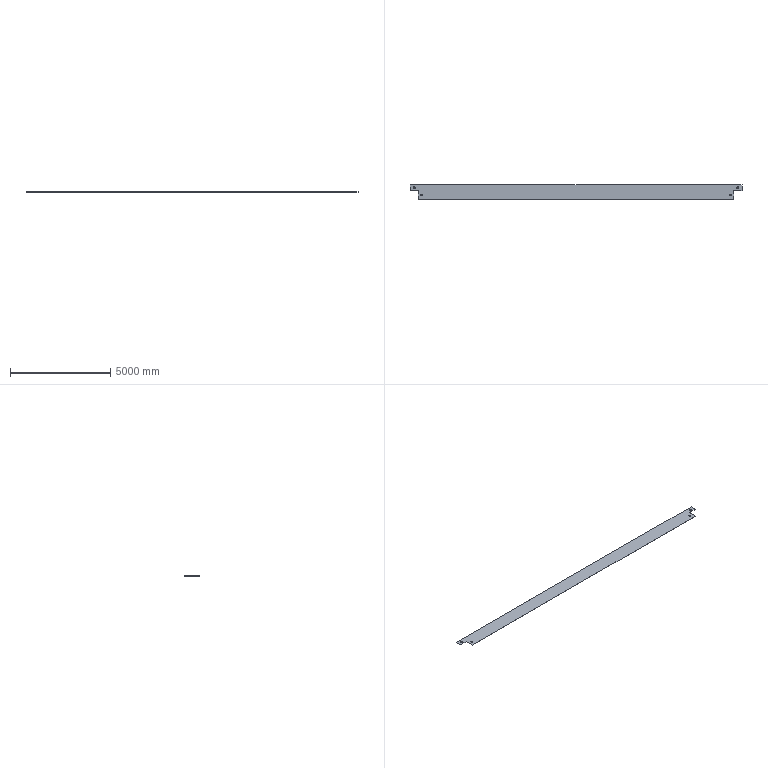Component | SolidWorks | SidePlate-1 | 1 solid | 18 faces | box 16570 x 748.03 x 6 mm | volume 70226722 mm3 | cylinder 10 | plane 8 | commonest cylinder face diameters 100 x8 3432081.25 x1 3440371.25 x1 | material Plain Carbon Steel
STEP:
#1=COLOUR_RGB('',0.7922,0.8196,0.9333);
#2=FILL_AREA_STYLE_COLOUR('',#1);
#3=FILL_AREA_STYLE('',(#2));
#4=SURFACE_STYLE_FILL_AREA(#3);
#5=SURFACE_SIDE_STYLE('',(#4));
#6=SURFACE_STYLE_USAGE(.BOTH.,#5);
#7=PRESENTATION_STYLE_ASSIGNMENT((#6));
#8=CARTESIAN_POINT('',(662.793,122.63,79.696));
#9=VERTEX_POINT('',#8);
#10=CARTESIAN_POINT('',(662.793,118.693,79.696));
#11=VERTEX_POINT('',#10);
#12=CARTESIAN_POINT('',(662.793,120.662,79.696));
#13=DIRECTION('',(0.,-0.,1.));
#14=DIRECTION('',(0.,1.,0.));
#15=AXIS2_PLACEMENT_3D('',#12,#13,#14);
#16=CIRCLE('',#15,1.969);
#17=EDGE_CURVE('',#9,#11,#16,.T.);
#18=ORIENTED_EDGE('',*,*,#17,.F.);
#19=CARTESIAN_POINT('',(662.793,122.63,79.933));
#20=VERTEX_POINT('',#19);
#21=CARTESIAN_POINT('',(662.793,122.63,79.696));
#22=DIRECTION('',(0.,-0.,1.));
#23=VECTOR('',#22,39.37);
#24=LINE('',#21,#23);
#25=EDGE_CURVE('',#9,#20,#24,.T.);
#26=ORIENTED_EDGE('',*,*,#25,.T.);
#27=CARTESIAN_POINT('',(662.793,118.693,79.933));
#28=VERTEX_POINT('',#27);
#29=CARTESIAN_POINT('',(662.793,120.662,79.933));
#30=DIRECTION('',(0.,-0.,1.));
#31=DIRECTION('',(0.,1.,0.));
#32=AXIS2_PLACEMENT_3D('',#29,#30,#31);
#33=CIRCLE('',#32,1.969);
#34=EDGE_CURVE('',#20,#28,#33,.T.);
#35=ORIENTED_EDGE('',*,*,#34,.T.);
#36=CARTESIAN_POINT('',(662.793,118.693,79.696));
#37=DIRECTION('',(0.,-0.,1.));
#38=VECTOR('',#37,39.37);
#39=LINE('',#36,#38);
#40=EDGE_CURVE('',#11,#28,#39,.T.);
#41=ORIENTED_EDGE('',*,*,#40,.F.);
#42=EDGE_LOOP('',(#18,#26,#35,#41));
#43=FACE_OUTER_BOUND('',#42,.T.);
#44=CARTESIAN_POINT('',(662.793,120.662,79.696));
#45=DIRECTION('',(0.,-0.,1.));
#46=DIRECTION('',(0.,-1.,0.));
#47=AXIS2_PLACEMENT_3D('',#44,#45,#46);
#48=CYLINDRICAL_SURFACE('',#47,1.969);
#49=ADVANCED_FACE('',(#43),#48,.F.);
#50=CARTESIAN_POINT('',(647.832,108.26,79.696));
#51=VERTEX_POINT('',#50);
#52=CARTESIAN_POINT('',(647.832,104.323,79.696));
#53=VERTEX_POINT('',#52);
#54=CARTESIAN_POINT('',(647.832,106.291,79.696));
#55=DIRECTION('',(0.,-0.,1.));
#56=DIRECTION('',(0.,1.,0.));
#57=AXIS2_PLACEMENT_3D('',#54,#55,#56);
#58=CIRCLE('',#57,1.969);
#59=EDGE_CURVE('',#51,#53,#58,.T.);
#60=ORIENTED_EDGE('',*,*,#59,.F.);
#61=CARTESIAN_POINT('',(647.832,108.26,79.933));
#62=VERTEX_POINT('',#61);
#63=CARTESIAN_POINT('',(647.832,108.26,79.696));
#64=DIRECTION('',(0.,-0.,1.));
#65=VECTOR('',#64,39.37);
#66=LINE('',#63,#65);
#67=EDGE_CURVE('',#51,#62,#66,.T.);
#68=ORIENTED_EDGE('',*,*,#67,.T.);
#69=CARTESIAN_POINT('',(647.832,104.323,79.933));
#70=VERTEX_POINT('',#69);
#71=CARTESIAN_POINT('',(647.832,106.291,79.933));
#72=DIRECTION('',(0.,-0.,1.));
#73=DIRECTION('',(0.,1.,0.));
#74=AXIS2_PLACEMENT_3D('',#71,#72,#73);
#75=CIRCLE('',#74,1.969);
#76=EDGE_CURVE('',#62,#70,#75,.T.);
#77=ORIENTED_EDGE('',*,*,#76,.T.);
#78=CARTESIAN_POINT('',(647.832,104.323,79.696));
#79=DIRECTION('',(0.,-0.,1.));
#80=VECTOR('',#79,39.37);
#81=LINE('',#78,#80);
#82=EDGE_CURVE('',#53,#70,#81,.T.);
#83=ORIENTED_EDGE('',*,*,#82,.F.);
#84=EDGE_LOOP('',(#60,#68,#77,#83));
#85=FACE_OUTER_BOUND('',#84,.T.);
#86=CARTESIAN_POINT('',(647.832,106.291,79.696));
#87=DIRECTION('',(0.,-0.,1.));
#88=DIRECTION('',(0.,-1.,0.));
#89=AXIS2_PLACEMENT_3D('',#86,#87,#88);
#90=CYLINDRICAL_SURFACE('',#89,1.969);
#91=ADVANCED_FACE('',(#85),#90,.F.);
#92=CARTESIAN_POINT('',(41.927,108.26,79.696));
#93=VERTEX_POINT('',#92);
#94=CARTESIAN_POINT('',(41.927,104.323,79.696));
#95=VERTEX_POINT('',#94);
#96=CARTESIAN_POINT('',(41.927,106.291,79.696));
#97=DIRECTION('',(0.,-0.,1.));
#98=DIRECTION('',(0.,-1.,0.));
#99=AXIS2_PLACEMENT_3D('',#96,#97,#98);
#100=CIRCLE('',#99,1.969);
#101=EDGE_CURVE('',#93,#95,#100,.T.);
#102=ORIENTED_EDGE('',*,*,#101,.F.);
#103=CARTESIAN_POINT('',(41.927,108.26,79.933));
#104=VERTEX_POINT('',#103);
#105=CARTESIAN_POINT('',(41.927,108.26,79.696));
#106=DIRECTION('',(0.,-0.,1.));
#107=VECTOR('',#106,39.37);
#108=LINE('',#105,#107);
#109=EDGE_CURVE('',#93,#104,#108,.T.);
#110=ORIENTED_EDGE('',*,*,#109,.T.);
#111=CARTESIAN_POINT('',(41.927,104.323,79.933));
#112=VERTEX_POINT('',#111);
#113=CARTESIAN_POINT('',(41.927,106.291,79.933));
#114=DIRECTION('',(0.,-0.,1.));
#115=DIRECTION('',(0.,-1.,0.));
#116=AXIS2_PLACEMENT_3D('',#113,#114,#115);
#117=CIRCLE('',#116,1.969);
#118=EDGE_CURVE('',#104,#112,#117,.T.);
#119=ORIENTED_EDGE('',*,*,#118,.T.);
#120=CARTESIAN_POINT('',(41.927,104.323,79.696));
#121=DIRECTION('',(0.,-0.,1.));
#122=VECTOR('',#121,39.37);
#123=LINE('',#120,#122);
#124=EDGE_CURVE('',#95,#112,#123,.T.);
#125=ORIENTED_EDGE('',*,*,#124,.F.);
#126=EDGE_LOOP('',(#102,#110,#119,#125));
#127=FACE_OUTER_BOUND('',#126,.T.);
#128=CARTESIAN_POINT('',(41.927,106.291,79.696));
#129=DIRECTION('',(0.,-0.,1.));
#130=DIRECTION('',(0.,-1.,0.));
#131=AXIS2_PLACEMENT_3D('',#128,#129,#130);
#132=CYLINDRICAL_SURFACE('',#131,1.969);
#133=ADVANCED_FACE('',(#127),#132,.F.);
#134=CARTESIAN_POINT('',(26.966,122.63,79.696));
#135=VERTEX_POINT('',#134);
#136=CARTESIAN_POINT('',(26.966,118.693,79.696));
#137=VERTEX_POINT('',#136);
#138=CARTESIAN_POINT('',(26.966,120.662,79.696));
#139=DIRECTION('',(0.,-0.,1.));
#140=DIRECTION('',(0.,-1.,0.));
#141=AXIS2_PLACEMENT_3D('',#138,#139,#140);
#142=CIRCLE('',#141,1.969);
#143=EDGE_CURVE('',#135,#137,#142,.T.);
#144=ORIENTED_EDGE('',*,*,#143,.F.);
#145=CARTESIAN_POINT('',(26.966,122.63,79.933));
#146=VERTEX_POINT('',#145);
#147=CARTESIAN_POINT('',(26.966,122.63,79.696));
#148=DIRECTION('',(0.,-0.,1.));
#149=VECTOR('',#148,39.37);
#150=LINE('',#147,#149);
#151=EDGE_CURVE('',#135,#146,#150,.T.);
#152=ORIENTED_EDGE('',*,*,#151,.T.);
#153=CARTESIAN_POINT('',(26.966,118.693,79.933));
#154=VERTEX_POINT('',#153);
#155=CARTESIAN_POINT('',(26.966,120.662,79.933));
#156=DIRECTION('',(0.,-0.,1.));
#157=DIRECTION('',(0.,-1.,0.));
#158=AXIS2_PLACEMENT_3D('',#155,#156,#157);
#159=CIRCLE('',#158,1.969);
#160=EDGE_CURVE('',#146,#154,#159,.T.);
#161=ORIENTED_EDGE('',*,*,#160,.T.);
#162=CARTESIAN_POINT('',(26.966,118.693,79.696));
#163=DIRECTION('',(0.,-0.,1.));
#164=VECTOR('',#163,39.37);
#165=LINE('',#162,#164);
#166=EDGE_CURVE('',#137,#154,#165,.T.);
#167=ORIENTED_EDGE('',*,*,#166,.F.);
#168=EDGE_LOOP('',(#144,#152,#161,#167));
#169=FACE_OUTER_BOUND('',#168,.T.);
#170=CARTESIAN_POINT('',(26.966,120.662,79.696));
#171=DIRECTION('',(0.,-0.,1.));
#172=DIRECTION('',(0.,-1.,0.));
#173=AXIS2_PLACEMENT_3D('',#170,#171,#172);
#174=CYLINDRICAL_SURFACE('',#173,1.969);
#175=ADVANCED_FACE('',(#169),#174,.F.);
#176=CARTESIAN_POINT('',(671.061,126.37,79.933));
#177=VERTEX_POINT('',#176);
#178=CARTESIAN_POINT('',(18.698,126.37,79.933));
#179=VERTEX_POINT('',#178);
#180=CARTESIAN_POINT('',(344.879,-67433.497,79.933));
#181=DIRECTION('',(0.,-0.,1.));
#182=DIRECTION('',(0.,1.,0.));
#183=AXIS2_PLACEMENT_3D('',#180,#181,#182);
#184=CIRCLE('',#183,67560.655);
#185=EDGE_CURVE('',#177,#179,#184,.T.);
#186=ORIENTED_EDGE('',*,*,#185,.F.);
#187=CARTESIAN_POINT('',(671.061,126.37,79.696));
#188=VERTEX_POINT('',#187);
#189=CARTESIAN_POINT('',(671.061,126.37,79.696));
#190=DIRECTION('',(0.,-0.,1.));
#191=VECTOR('',#190,39.37);
#192=LINE('',#189,#191);
#193=EDGE_CURVE('',#188,#177,#192,.T.);
#194=ORIENTED_EDGE('',*,*,#193,.F.);
#195=CARTESIAN_POINT('',(18.698,126.37,79.696));
#196=VERTEX_POINT('',#195);
#197=CARTESIAN_POINT('',(344.879,-67433.497,79.696));
#198=DIRECTION('',(0.,-0.,1.));
#199=DIRECTION('',(0.,1.,0.));
#200=AXIS2_PLACEMENT_3D('',#197,#198,#199);
#201=CIRCLE('',#200,67560.655);
#202=EDGE_CURVE('',#188,#196,#201,.T.);
#203=ORIENTED_EDGE('',*,*,#202,.T.);
#204=CARTESIAN_POINT('',(18.698,126.37,79.696));
#205=DIRECTION('',(0.,-0.,1.));
#206=VECTOR('',#205,39.37);
#207=LINE('',#204,#206);
#208=EDGE_CURVE('',#196,#179,#207,.T.);
#209=ORIENTED_EDGE('',*,*,#208,.T.);
#210=EDGE_LOOP('',(#186,#194,#203,#209));
#211=FACE_OUTER_BOUND('',#210,.T.);
#212=CARTESIAN_POINT('',(344.879,-67433.497,79.696));
#213=DIRECTION('',(0.,-0.,1.));
#214=DIRECTION('',(0.,-1.,-0.));
#215=AXIS2_PLACEMENT_3D('',#212,#213,#214);
#216=CYLINDRICAL_SURFACE('',#215,67560.655);
#217=ADVANCED_FACE('',(#211),#216,.T.);
#218=CARTESIAN_POINT('',(671.061,114.953,79.933));
#219=VERTEX_POINT('',#218);
#220=CARTESIAN_POINT('',(671.061,114.953,79.933));
#221=DIRECTION('',(0.,1.,0.));
#222=VECTOR('',#221,39.37);
#223=LINE('',#220,#222);
#224=EDGE_CURVE('',#219,#177,#223,.T.);
#225=ORIENTED_EDGE('',*,*,#224,.F.);
#226=CARTESIAN_POINT('',(671.061,114.953,79.696));
#227=VERTEX_POINT('',#226);
#228=CARTESIAN_POINT('',(671.061,114.953,79.696));
#229=DIRECTION('',(0.,-0.,1.));
#230=VECTOR('',#229,39.37);
#231=LINE('',#228,#230);
#232=EDGE_CURVE('',#227,#219,#231,.T.);
#233=ORIENTED_EDGE('',*,*,#232,.F.);
#234=CARTESIAN_POINT('',(671.061,114.953,79.696));
#235=DIRECTION('',(0.,1.,0.));
#236=VECTOR('',#235,39.37);
#237=LINE('',#234,#236);
#238=EDGE_CURVE('',#227,#188,#237,.T.);
#239=ORIENTED_EDGE('',*,*,#238,.T.);
#240=ORIENTED_EDGE('',*,*,#193,.T.);
#241=EDGE_LOOP('',(#225,#233,#239,#240));
#242=FACE_OUTER_BOUND('',#241,.T.);
#243=CARTESIAN_POINT('',(671.061,114.953,79.696));
#244=DIRECTION('',(1.,0.,0.));
#245=DIRECTION('',(0.,1.,0.));
#246=AXIS2_PLACEMENT_3D('',#243,#244,#245);
#247=PLANE('',#246);
#248=ADVANCED_FACE('',(#242),#247,.T.);
#249=CARTESIAN_POINT('',(654.919,114.953,79.933));
#250=VERTEX_POINT('',#249);
#251=CARTESIAN_POINT('',(671.061,114.953,79.933));
#252=DIRECTION('',(1.,0.,0.));
#253=VECTOR('',#252,39.37);
#254=LINE('',#251,#253);
#255=EDGE_CURVE('',#250,#219,#254,.T.);
#256=ORIENTED_EDGE('',*,*,#255,.F.);
#257=CARTESIAN_POINT('',(654.919,114.953,79.696));
#258=VERTEX_POINT('',#257);
#259=CARTESIAN_POINT('',(654.919,114.953,79.696));
#260=DIRECTION('',(0.,-0.,1.));
#261=VECTOR('',#260,39.37);
#262=LINE('',#259,#261);
#263=EDGE_CURVE('',#258,#250,#262,.T.);
#264=ORIENTED_EDGE('',*,*,#263,.F.);
#265=CARTESIAN_POINT('',(671.061,114.953,79.696));
#266=DIRECTION('',(1.,0.,0.));
#267=VECTOR('',#266,39.37);
#268=LINE('',#265,#267);
#269=EDGE_CURVE('',#258,#227,#268,.T.);
#270=ORIENTED_EDGE('',*,*,#269,.T.);
#271=ORIENTED_EDGE('',*,*,#232,.T.);
#272=EDGE_LOOP('',(#256,#264,#270,#271));
#273=FACE_OUTER_BOUND('',#272,.T.);
#274=CARTESIAN_POINT('',(671.061,114.953,79.696));
#275=DIRECTION('',(0.,-1.,-0.));
#276=DIRECTION('',(1.,0.,0.));
#277=AXIS2_PLACEMENT_3D('',#274,#275,#276);
#278=PLANE('',#277);
#279=ADVANCED_FACE('',(#273),#278,.T.);
#280=CARTESIAN_POINT('',(654.919,97.708,79.933));
#281=VERTEX_POINT('',#280);
#282=CARTESIAN_POINT('',(654.919,114.953,79.933));
#283=DIRECTION('',(0.,1.,0.));
#284=VECTOR('',#283,39.37);
#285=LINE('',#282,#284);
#286=EDGE_CURVE('',#281,#250,#285,.T.);
#287=ORIENTED_EDGE('',*,*,#286,.F.);
#288=CARTESIAN_POINT('',(654.919,97.708,79.696));
#289=VERTEX_POINT('',#288);
#290=CARTESIAN_POINT('',(654.919,97.708,79.696));
#291=DIRECTION('',(0.,-0.,1.));
#292=VECTOR('',#291,39.37);
#293=LINE('',#290,#292);
#294=EDGE_CURVE('',#289,#281,#293,.T.);
#295=ORIENTED_EDGE('',*,*,#294,.F.);
#296=CARTESIAN_POINT('',(654.919,114.953,79.696));
#297=DIRECTION('',(0.,1.,0.));
#298=VECTOR('',#297,39.37);
#299=LINE('',#296,#298);
#300=EDGE_CURVE('',#289,#258,#299,.T.);
#301=ORIENTED_EDGE('',*,*,#300,.T.);
#302=ORIENTED_EDGE('',*,*,#263,.T.);
#303=EDGE_LOOP('',(#287,#295,#301,#302));
#304=FACE_OUTER_BOUND('',#303,.T.);
#305=CARTESIAN_POINT('',(654.919,114.953,79.696));
#306=DIRECTION('',(1.,0.,0.));
#307=DIRECTION('',(0.,1.,0.));
#308=AXIS2_PLACEMENT_3D('',#305,#306,#307);
#309=PLANE('',#308);
#310=ADVANCED_FACE('',(#304),#309,.T.);
#311=CARTESIAN_POINT('',(34.84,97.708,79.933));
#312=VERTEX_POINT('',#311);
#313=CARTESIAN_POINT('',(344.879,-67625.426,79.933));
#314=DIRECTION('',(0.,0.,-1.));
#315=DIRECTION('',(0.,1.,0.));
#316=AXIS2_PLACEMENT_3D('',#313,#314,#315);
#317=CIRCLE('',#316,67723.844);
#318=EDGE_CURVE('',#312,#281,#317,.T.);
#319=ORIENTED_EDGE('',*,*,#318,.F.);
#320=CARTESIAN_POINT('',(34.84,97.708,79.696));
#321=VERTEX_POINT('',#320);
#322=CARTESIAN_POINT('',(34.84,97.708,79.696));
#323=DIRECTION('',(0.,-0.,1.));
#324=VECTOR('',#323,39.37);
#325=LINE('',#322,#324);
#326=EDGE_CURVE('',#321,#312,#325,.T.);
#327=ORIENTED_EDGE('',*,*,#326,.F.);
#328=CARTESIAN_POINT('',(344.879,-67625.426,79.696));
#329=DIRECTION('',(0.,0.,-1.));
#330=DIRECTION('',(0.,1.,0.));
#331=AXIS2_PLACEMENT_3D('',#328,#329,#330);
#332=CIRCLE('',#331,67723.844);
#333=EDGE_CURVE('',#321,#289,#332,.T.);
#334=ORIENTED_EDGE('',*,*,#333,.T.);
#335=ORIENTED_EDGE('',*,*,#294,.T.);
#336=EDGE_LOOP('',(#319,#327,#334,#335));
#337=FACE_OUTER_BOUND('',#336,.T.);
#338=CARTESIAN_POINT('',(344.879,-67625.426,79.696));
#339=DIRECTION('',(0.,-0.,1.));
#340=DIRECTION('',(0.,-1.,-0.));
#341=AXIS2_PLACEMENT_3D('',#338,#339,#340);
#342=CYLINDRICAL_SURFACE('',#341,67723.844);
#343=ADVANCED_FACE('',(#337),#342,.F.);
#344=CARTESIAN_POINT('',(34.84,114.953,79.933));
#345=VERTEX_POINT('',#344);
#346=CARTESIAN_POINT('',(34.84,114.953,79.933));
#347=DIRECTION('',(0.,-1.,-0.));
#348=VECTOR('',#347,39.37);
#349=LINE('',#346,#348);
#350=EDGE_CURVE('',#345,#312,#349,.T.);
#351=ORIENTED_EDGE('',*,*,#350,.F.);
#352=CARTESIAN_POINT('',(34.84,114.953,79.696));
#353=VERTEX_POINT('',#352);
#354=CARTESIAN_POINT('',(34.84,114.953,79.696));
#355=DIRECTION('',(0.,-0.,1.));
#356=VECTOR('',#355,39.37);
#357=LINE('',#354,#356);
#358=EDGE_CURVE('',#353,#345,#357,.T.);
#359=ORIENTED_EDGE('',*,*,#358,.F.);
#360=CARTESIAN_POINT('',(34.84,114.953,79.696));
#361=DIRECTION('',(0.,-1.,-0.));
#362=VECTOR('',#361,39.37);
#363=LINE('',#360,#362);
#364=EDGE_CURVE('',#353,#321,#363,.T.);
#365=ORIENTED_EDGE('',*,*,#364,.T.);
#366=ORIENTED_EDGE('',*,*,#326,.T.);
#367=EDGE_LOOP('',(#351,#359,#365,#366));
#368=FACE_OUTER_BOUND('',#367,.T.);
#369=CARTESIAN_POINT('',(34.84,114.953,79.696));
#370=DIRECTION('',(-1.,-0.,-0.));
#371=DIRECTION('',(0.,-1.,-0.));
#372=AXIS2_PLACEMENT_3D('',#369,#370,#371);
#373=PLANE('',#372);
#374=ADVANCED_FACE('',(#368),#373,.T.);
#375=CARTESIAN_POINT('',(18.698,114.953,79.933));
#376=VERTEX_POINT('',#375);
#377=CARTESIAN_POINT('',(18.698,114.953,79.933));
#378=DIRECTION('',(1.,0.,0.));
#379=VECTOR('',#378,39.37);
#380=LINE('',#377,#379);
#381=EDGE_CURVE('',#376,#345,#380,.T.);
#382=ORIENTED_EDGE('',*,*,#381,.F.);
#383=CARTESIAN_POINT('',(18.698,114.953,79.696));
#384=VERTEX_POINT('',#383);
#385=CARTESIAN_POINT('',(18.698,114.953,79.696));
#386=DIRECTION('',(0.,-0.,1.));
#387=VECTOR('',#386,39.37);
#388=LINE('',#385,#387);
#389=EDGE_CURVE('',#384,#376,#388,.T.);
#390=ORIENTED_EDGE('',*,*,#389,.F.);
#391=CARTESIAN_POINT('',(18.698,114.953,79.696));
#392=DIRECTION('',(1.,0.,0.));
#393=VECTOR('',#392,39.37);
#394=LINE('',#391,#393);
#395=EDGE_CURVE('',#384,#353,#394,.T.);
#396=ORIENTED_EDGE('',*,*,#395,.T.);
#397=ORIENTED_EDGE('',*,*,#358,.T.);
#398=EDGE_LOOP('',(#382,#390,#396,#397));
#399=FACE_OUTER_BOUND('',#398,.T.);
#400=CARTESIAN_POINT('',(18.698,114.953,79.696));
#401=DIRECTION('',(0.,-1.,-0.));
#402=DIRECTION('',(1.,0.,0.));
#403=AXIS2_PLACEMENT_3D('',#400,#401,#402);
#404=PLANE('',#403);
#405=ADVANCED_FACE('',(#399),#404,.T.);
#406=CARTESIAN_POINT('',(18.698,126.37,79.933));
#407=DIRECTION('',(0.,-1.,-0.));
#408=VECTOR('',#407,39.37);
#409=LINE('',#406,#408);
#410=EDGE_CURVE('',#179,#376,#409,.T.);
#411=ORIENTED_EDGE('',*,*,#410,.F.);
#412=ORIENTED_EDGE('',*,*,#208,.F.);
#413=CARTESIAN_POINT('',(18.698,126.37,79.696));
#414=DIRECTION('',(0.,-1.,-0.));
#415=VECTOR('',#414,39.37);
#416=LINE('',#413,#415);
#417=EDGE_CURVE('',#196,#384,#416,.T.);
#418=ORIENTED_EDGE('',*,*,#417,.T.);
#419=ORIENTED_EDGE('',*,*,#389,.T.);
#420=EDGE_LOOP('',(#411,#412,#418,#419));
#421=FACE_OUTER_BOUND('',#420,.T.);
#422=CARTESIAN_POINT('',(18.698,126.37,79.696));
#423=DIRECTION('',(-1.,-0.,-0.));
#424=DIRECTION('',(0.,-1.,-0.));
#425=AXIS2_PLACEMENT_3D('',#422,#423,#424);
#426=PLANE('',#425);
#427=ADVANCED_FACE('',(#421),#426,.T.);
#428=CARTESIAN_POINT('',(662.793,120.662,79.696));
#429=DIRECTION('',(0.,-0.,1.));
#430=DIRECTION('',(0.,1.,0.));
#431=AXIS2_PLACEMENT_3D('',#428,#429,#430);
#432=CIRCLE('',#431,1.969);
#433=EDGE_CURVE('',#11,#9,#432,.T.);
#434=ORIENTED_EDGE('',*,*,#433,.T.);
#435=ORIENTED_EDGE('',*,*,#17,.T.);
#436=EDGE_LOOP('',(#434,#435));
#437=FACE_BOUND('',#436,.T.);
#438=CARTESIAN_POINT('',(647.832,106.291,79.696));
#439=DIRECTION('',(0.,-0.,1.));
#440=DIRECTION('',(0.,1.,0.));
#441=AXIS2_PLACEMENT_3D('',#438,#439,#440);
#442=CIRCLE('',#441,1.969);
#443=EDGE_CURVE('',#53,#51,#442,.T.);
#444=ORIENTED_EDGE('',*,*,#443,.T.);
#445=ORIENTED_EDGE('',*,*,#59,.T.);
#446=EDGE_LOOP('',(#444,#445));
#447=FACE_BOUND('',#446,.T.);
#448=CARTESIAN_POINT('',(41.927,106.291,79.696));
#449=DIRECTION('',(0.,-0.,1.));
#450=DIRECTION('',(0.,-1.,0.));
#451=AXIS2_PLACEMENT_3D('',#448,#449,#450);
#452=CIRCLE('',#451,1.969);
#453=EDGE_CURVE('',#95,#93,#452,.T.);
#454=ORIENTED_EDGE('',*,*,#453,.T.);
#455=ORIENTED_EDGE('',*,*,#101,.T.);
#456=EDGE_LOOP('',(#454,#455));
#457=FACE_BOUND('',#456,.T.);
#458=CARTESIAN_POINT('',(26.966,120.662,79.696));
#459=DIRECTION('',(0.,-0.,1.));
#460=DIRECTION('',(0.,-1.,0.));
#461=AXIS2_PLACEMENT_3D('',#458,#459,#460);
#462=CIRCLE('',#461,1.969);
#463=EDGE_CURVE('',#137,#135,#462,.T.);
#464=ORIENTED_EDGE('',*,*,#463,.T.);
#465=ORIENTED_EDGE('',*,*,#143,.T.);
#466=EDGE_LOOP('',(#464,#465));
#467=FACE_BOUND('',#466,.T.);
#468=ORIENTED_EDGE('',*,*,#202,.F.);
#469=ORIENTED_EDGE('',*,*,#238,.F.);
#470=ORIENTED_EDGE('',*,*,#269,.F.);
#471=ORIENTED_EDGE('',*,*,#300,.F.);
#472=ORIENTED_EDGE('',*,*,#333,.F.);
#473=ORIENTED_EDGE('',*,*,#364,.F.);
#474=ORIENTED_EDGE('',*,*,#395,.F.);
#475=ORIENTED_EDGE('',*,*,#417,.F.);
#476=EDGE_LOOP('',(#468,#469,#470,#471,#472,#473,#474,#475));
#477=FACE_OUTER_BOUND('',#476,.T.);
#478=CARTESIAN_POINT('',(344.879,-67433.497,79.696));
#479=DIRECTION('',(0.,0.,-1.));
#480=DIRECTION('',(0.,1.,0.));
#481=AXIS2_PLACEMENT_3D('',#478,#479,#480);
#482=PLANE('',#481);
#483=ADVANCED_FACE('',(#437,#447,#457,#467,#477),#482,.T.);
#484=CARTESIAN_POINT('',(662.793,120.662,79.933));
#485=DIRECTION('',(0.,-0.,1.));
#486=DIRECTION('',(0.,1.,0.));
#487=AXIS2_PLACEMENT_3D('',#484,#485,#486);
#488=CIRCLE('',#487,1.969);
#489=EDGE_CURVE('',#28,#20,#488,.T.);
#490=ORIENTED_EDGE('',*,*,#489,.F.);
#491=ORIENTED_EDGE('',*,*,#34,.F.);
#492=EDGE_LOOP('',(#490,#491));
#493=FACE_BOUND('',#492,.T.);
#494=CARTESIAN_POINT('',(647.832,106.291,79.933));
#495=DIRECTION('',(0.,-0.,1.));
#496=DIRECTION('',(0.,1.,0.));
#497=AXIS2_PLACEMENT_3D('',#494,#495,#496);
#498=CIRCLE('',#497,1.969);
#499=EDGE_CURVE('',#70,#62,#498,.T.);
#500=ORIENTED_EDGE('',*,*,#499,.F.);
#501=ORIENTED_EDGE('',*,*,#76,.F.);
#502=EDGE_LOOP('',(#500,#501));
#503=FACE_BOUND('',#502,.T.);
#504=CARTESIAN_POINT('',(41.927,106.291,79.933));
#505=DIRECTION('',(0.,-0.,1.));
#506=DIRECTION('',(0.,-1.,0.));
#507=AXIS2_PLACEMENT_3D('',#504,#505,#506);
#508=CIRCLE('',#507,1.969);
#509=EDGE_CURVE('',#112,#104,#508,.T.);
#510=ORIENTED_EDGE('',*,*,#509,.F.);
#511=ORIENTED_EDGE('',*,*,#118,.F.);
#512=EDGE_LOOP('',(#510,#511));
#513=FACE_BOUND('',#512,.T.);
#514=CARTESIAN_POINT('',(26.966,120.662,79.933));
#515=DIRECTION('',(0.,-0.,1.));
#516=DIRECTION('',(0.,-1.,0.));
#517=AXIS2_PLACEMENT_3D('',#514,#515,#516);
#518=CIRCLE('',#517,1.969);
#519=EDGE_CURVE('',#154,#146,#518,.T.);
#520=ORIENTED_EDGE('',*,*,#519,.F.);
#521=ORIENTED_EDGE('',*,*,#160,.F.);
#522=EDGE_LOOP('',(#520,#521));
#523=FACE_BOUND('',#522,.T.);
#524=ORIENTED_EDGE('',*,*,#185,.T.);
#525=ORIENTED_EDGE('',*,*,#410,.T.);
#526=ORIENTED_EDGE('',*,*,#381,.T.);
#527=ORIENTED_EDGE('',*,*,#350,.T.);
#528=ORIENTED_EDGE('',*,*,#318,.T.);
#529=ORIENTED_EDGE('',*,*,#286,.T.);
#530=ORIENTED_EDGE('',*,*,#255,.T.);
#531=ORIENTED_EDGE('',*,*,#224,.T.);
#532=EDGE_LOOP('',(#524,#525,#526,#527,#528,#529,#530,#531));
#533=FACE_OUTER_BOUND('',#532,.T.);
#534=CARTESIAN_POINT('',(344.879,-67433.497,79.933));
#535=DIRECTION('',(0.,0.,-1.));
#536=DIRECTION('',(0.,1.,0.));
#537=AXIS2_PLACEMENT_3D('',#534,#535,#536);
#538=PLANE('',#537);
#539=ADVANCED_FACE('',(#493,#503,#513,#523,#533),#538,.F.);
#540=ORIENTED_EDGE('',*,*,#151,.F.);
#541=ORIENTED_EDGE('',*,*,#463,.F.);
#542=ORIENTED_EDGE('',*,*,#166,.T.);
#543=ORIENTED_EDGE('',*,*,#519,.T.);
#544=EDGE_LOOP('',(#540,#541,#542,#543));
#545=FACE_OUTER_BOUND('',#544,.T.);
#546=CARTESIAN_POINT('',(26.966,120.662,79.696));
#547=DIRECTION('',(0.,-0.,1.));
#548=DIRECTION('',(0.,-1.,0.));
#549=AXIS2_PLACEMENT_3D('',#546,#547,#548);
#550=CYLINDRICAL_SURFACE('',#549,1.969);
#551=ADVANCED_FACE('',(#545),#550,.F.);
#552=ORIENTED_EDGE('',*,*,#109,.F.);
#553=ORIENTED_EDGE('',*,*,#453,.F.);
#554=ORIENTED_EDGE('',*,*,#124,.T.);
#555=ORIENTED_EDGE('',*,*,#509,.T.);
#556=EDGE_LOOP('',(#552,#553,#554,#555));
#557=FACE_OUTER_BOUND('',#556,.T.);
#558=CARTESIAN_POINT('',(41.927,106.291,79.696));
#559=DIRECTION('',(0.,-0.,1.));
#560=DIRECTION('',(0.,-1.,0.));
#561=AXIS2_PLACEMENT_3D('',#558,#559,#560);
#562=CYLINDRICAL_SURFACE('',#561,1.969);
#563=ADVANCED_FACE('',(#557),#562,.F.);
#564=ORIENTED_EDGE('',*,*,#67,.F.);
#565=ORIENTED_EDGE('',*,*,#443,.F.);
#566=ORIENTED_EDGE('',*,*,#82,.T.);
#567=ORIENTED_EDGE('',*,*,#499,.T.);
#568=EDGE_LOOP('',(#564,#565,#566,#567));
#569=FACE_OUTER_BOUND('',#568,.T.);
#570=CARTESIAN_POINT('',(647.832,106.291,79.696));
#571=DIRECTION('',(0.,-0.,1.));
#572=DIRECTION('',(0.,-1.,0.));
#573=AXIS2_PLACEMENT_3D('',#570,#571,#572);
#574=CYLINDRICAL_SURFACE('',#573,1.969);
#575=ADVANCED_FACE('',(#569),#574,.F.);
#576=ORIENTED_EDGE('',*,*,#25,.F.);
#577=ORIENTED_EDGE('',*,*,#433,.F.);
#578=ORIENTED_EDGE('',*,*,#40,.T.);
#579=ORIENTED_EDGE('',*,*,#489,.T.);
#580=EDGE_LOOP('',(#576,#577,#578,#579));
#581=FACE_OUTER_BOUND('',#580,.T.);
#582=CARTESIAN_POINT('',(662.793,120.662,79.696));
#583=DIRECTION('',(0.,-0.,1.));
#584=DIRECTION('',(0.,-1.,0.));
#585=AXIS2_PLACEMENT_3D('',#582,#583,#584);
#586=CYLINDRICAL_SURFACE('',#585,1.969);
#587=ADVANCED_FACE('',(#581),#586,.F.);
#588=CLOSED_SHELL('',(#49,#91,#133,#175,#217,#248,#279,#310,#343,#374,#405,#427,#483,#539,#551,#563,#575,#587));
#589=MANIFOLD_SOLID_BREP('',#588);
#590=STYLED_ITEM('',(#7),#589);
#591=PRESENTATION_LAYER_ASSIGNMENT('','',(#590));
#592=CARTESIAN_POINT('',(0.,0.,0.));
#593=DIRECTION('',(0.,0.,1.));
#594=DIRECTION('',(1.,0.,0.));
#595=AXIS2_PLACEMENT_3D('',#592,#593,#594);
#596=(LENGTH_UNIT()NAMED_UNIT(*)SI_UNIT($,.METRE.));
#597=LENGTH_MEASURE_WITH_UNIT(LENGTH_MEASURE(0.0254),#596);
#598=DIMENSIONAL_EXPONENTS(1.,0.,0.,0.,0.,0.,0.);
#599=(CONVERSION_BASED_UNIT('',#597)LENGTH_UNIT()NAMED_UNIT(#598));
#600=UNCERTAINTY_MEASURE_WITH_UNIT(LENGTH_MEASURE(0.00001),#599,'','');
#601=(NAMED_UNIT(*)PLANE_ANGLE_UNIT()SI_UNIT($,.RADIAN.));
#602=(NAMED_UNIT(*)SI_UNIT($,.STERADIAN.)SOLID_ANGLE_UNIT());
#603=(GEOMETRIC_REPRESENTATION_CONTEXT(3)GLOBAL_UNCERTAINTY_ASSIGNED_CONTEXT((#600))GLOBAL_UNIT_ASSIGNED_CONTEXT((#599,#601,#602))REPRESENTATION_CONTEXT('',''));
#604=ADVANCED_BREP_SHAPE_REPRESENTATION('',(#589,#595),#603);
#605=(LENGTH_UNIT()NAMED_UNIT(*)SI_UNIT($,.METRE.));
#606=LENGTH_MEASURE_WITH_UNIT(LENGTH_MEASURE(0.0254),#605);
#607=DIMENSIONAL_EXPONENTS(1.,0.,0.,0.,0.,0.,0.);
#608=(CONVERSION_BASED_UNIT('',#606)LENGTH_UNIT()NAMED_UNIT(#607));
#609=UNCERTAINTY_MEASURE_WITH_UNIT(LENGTH_MEASURE(0.00001),#608,'','');
#610=(NAMED_UNIT(*)PLANE_ANGLE_UNIT()SI_UNIT($,.RADIAN.));
#611=(NAMED_UNIT(*)SI_UNIT($,.STERADIAN.)SOLID_ANGLE_UNIT());
#612=(GEOMETRIC_REPRESENTATION_CONTEXT(3)GLOBAL_UNCERTAINTY_ASSIGNED_CONTEXT((#609))GLOBAL_UNIT_ASSIGNED_CONTEXT((#608,#610,#611))REPRESENTATION_CONTEXT('',''));
#613=MECHANICAL_DESIGN_GEOMETRIC_PRESENTATION_REPRESENTATION('',(#590),#612);